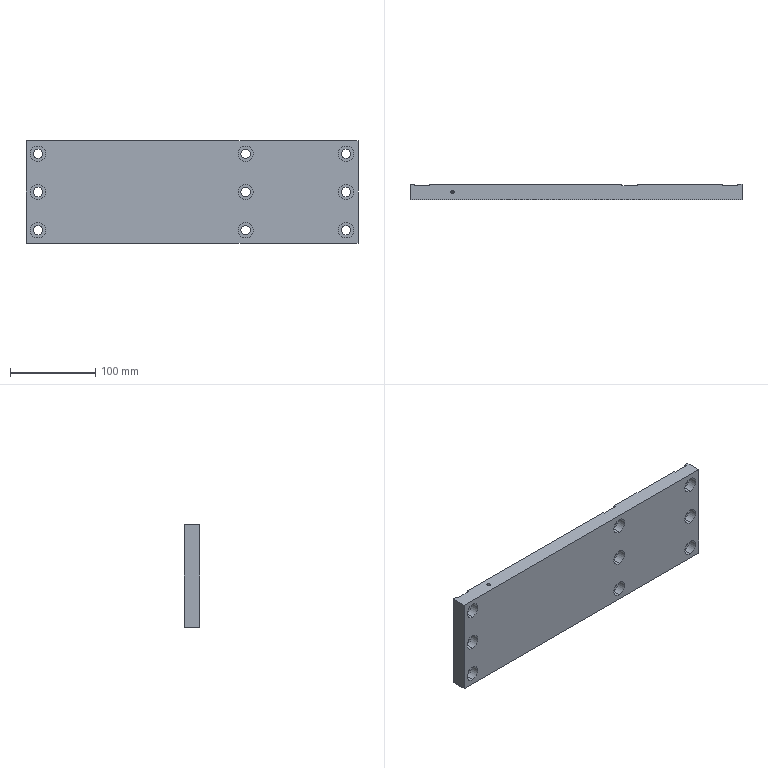Component | SolidWorks | ZL-11-01CoverPlate-1 | 1 solid | 71 faces | box 390 x 18 x 120 mm | volume 801051 mm3 | cylinder 40 | plane 27 | cone 4 | commonest cylinder face diameters 18 x18 11 x18 4.2 x4
build123d program:
from build123d import *

# Parameters (mm, degrees)
SKETCH1_W                                        = 390
SKETCH1_H                                        = 18
EXTRUDE1_DEPTH                                   = 60
SKETCH2_W                                        = 18
SKETCH2_H                                        = 2
CUT_EXTRUDE1_DEPTH                               = 409.441
M10_HEX_SOCKET_HEAD_CAP_SCREW_CBORE1_D           = 11
M10_HEX_SOCKET_HEAD_CAP_SCREW_CBORE1_CBORE_D     = 18
M10_HEX_SOCKET_HEAD_CAP_SCREW_CBORE1_CBORE_DEPTH = 10
LPATTERN1_COUNT                                  = 3
LPATTERN1_PITCH                                  = 45
LPATTERN2_COUNT                                  = 2
LPATTERN2_PITCH                                  = 118
LPATTERN2_COPY_1_D                               = 11
LPATTERN2_COPY_1_CBORE_D                         = 18
LPATTERN2_COPY_1_CBORE_DEPTH                     = 10
LPATTERN2_COPY_2_D                               = 11
LPATTERN2_COPY_2_CBORE_D                         = 18
LPATTERN2_COPY_2_CBORE_DEPTH                     = 10
LPATTERN3_COUNT                                  = 2
LPATTERN3_PITCH                                  = 362
LPATTERN3_COPY_1_D                               = 11
LPATTERN3_COPY_1_CBORE_D                         = 18
LPATTERN3_COPY_1_CBORE_DEPTH                     = 10
LPATTERN3_COPY_2_D                               = 11
LPATTERN3_COPY_2_CBORE_D                         = 18
LPATTERN3_COPY_2_CBORE_DEPTH                     = 10


with BuildPart() as part:
    # Sketch1 → Extrude1 (new, symmetric)
    with BuildSketch(Plane.XY):
        with Locations((-195, 9)):
            Rectangle(SKETCH1_W, SKETCH1_H)
    extrude(amount=EXTRUDE1_DEPTH, both=True)

    # Sketch2 → Cut-Extrude1 (cut, through all)
    with BuildSketch(Plane.XY.offset(60)):
        with Locations((-14, 17)):
            Rectangle(SKETCH2_W, SKETCH2_H)
    cut_extrude1 = extrude(amount=-CUT_EXTRUDE1_DEPTH, mode=Mode.SUBTRACT)

    # M10 Hex Socket Head Cap Screw CBORE1 (through all)
    with Locations(Plane(origin=(-2.151, 0, -37.249), x_dir=(-1, 0, 0), z_dir=(0, -1, 0))):
        with Locations((11.849, 7.751)):
            m10_hex_socket_head_cap_screw_cbore1 = CounterBoreHole(M10_HEX_SOCKET_HEAD_CAP_SCREW_CBORE1_D / 2, M10_HEX_SOCKET_HEAD_CAP_SCREW_CBORE1_CBORE_D / 2, M10_HEX_SOCKET_HEAD_CAP_SCREW_CBORE1_CBORE_DEPTH)

    # LPattern1: M10 Hex Socket Head Cap Screw CBORE1 ×3
    with Locations(*[(0, 0, i * LPATTERN1_PITCH) for i in range(1, LPATTERN1_COUNT)]):
        add(m10_hex_socket_head_cap_screw_cbore1, mode=Mode.SUBTRACT)

    # LPattern2: Cut-Extrude1, M10 Hex Socket Head Cap Screw CBORE1 ×2
    with Locations(*[(-i * LPATTERN2_PITCH, 0, 0) for i in range(1, LPATTERN2_COUNT)]):
        add(cut_extrude1, mode=Mode.SUBTRACT)
        add(m10_hex_socket_head_cap_screw_cbore1, mode=Mode.SUBTRACT)

    # LPattern2 copy 1 (through all)
    with Locations(Plane(origin=(-120.151, 0, 7.751), x_dir=(-1, 0, 0), z_dir=(0, -1, 0))):
        with Locations((11.849, 7.751)):
            CounterBoreHole(LPATTERN2_COPY_1_D / 2, LPATTERN2_COPY_1_CBORE_D / 2, LPATTERN2_COPY_1_CBORE_DEPTH)

    # LPattern2 copy 2 (through all)
    with Locations(Plane(origin=(-120.151, 0, 52.751), x_dir=(-1, 0, 0), z_dir=(0, -1, 0))):
        with Locations((11.849, 7.751)):
            CounterBoreHole(LPATTERN2_COPY_2_D / 2, LPATTERN2_COPY_2_CBORE_D / 2, LPATTERN2_COPY_2_CBORE_DEPTH)

    # LPattern3: Cut-Extrude1, M10 Hex Socket Head Cap Screw CBORE1 ×2
    with Locations(*[(-i * LPATTERN3_PITCH, 0, 0) for i in range(1, LPATTERN3_COUNT)]):
        add(cut_extrude1, mode=Mode.SUBTRACT)
        add(m10_hex_socket_head_cap_screw_cbore1, mode=Mode.SUBTRACT)

    # LPattern3 copy 1 (through all)
    with Locations(Plane(origin=(-364.151, 0, 7.751), x_dir=(-1, 0, 0), z_dir=(0, -1, 0))):
        with Locations((11.849, 7.751)):
            CounterBoreHole(LPATTERN3_COPY_1_D / 2, LPATTERN3_COPY_1_CBORE_D / 2, LPATTERN3_COPY_1_CBORE_DEPTH)

    # LPattern3 copy 2 (through all)
    with Locations(Plane(origin=(-364.151, 0, 52.751), x_dir=(-1, 0, 0), z_dir=(0, -1, 0))):
        with Locations((11.849, 7.751)):
            CounterBoreHole(LPATTERN3_COPY_2_D / 2, LPATTERN3_COPY_2_CBORE_D / 2, LPATTERN3_COPY_2_CBORE_DEPTH)

    # Sketch5 → M5 Tapped Hole1 (revolve, cut)
    with BuildSketch(Plane(origin=(-340, 9, -60), x_dir=(0, 1, 0), z_dir=(1, 0, 0))):
        Polygon((0, 0), (0, 13.662), (2.1, 12.4), (2.1, 0), align=None)
    m5_tapped_hole1 = revolve(axis=Axis((-340, 9, -66.35), (0, 0, 1)), mode=Mode.SUBTRACT)

    # Mirror1: M5 Tapped Hole1 across plane
    add(m5_tapped_hole1.mirror(Plane.XY), mode=Mode.SUBTRACT)


solid = part.part

# Placed as in the assembly
solid = solid.moved(Location((198.552, 38.22, 0), (0, 0, 0)))